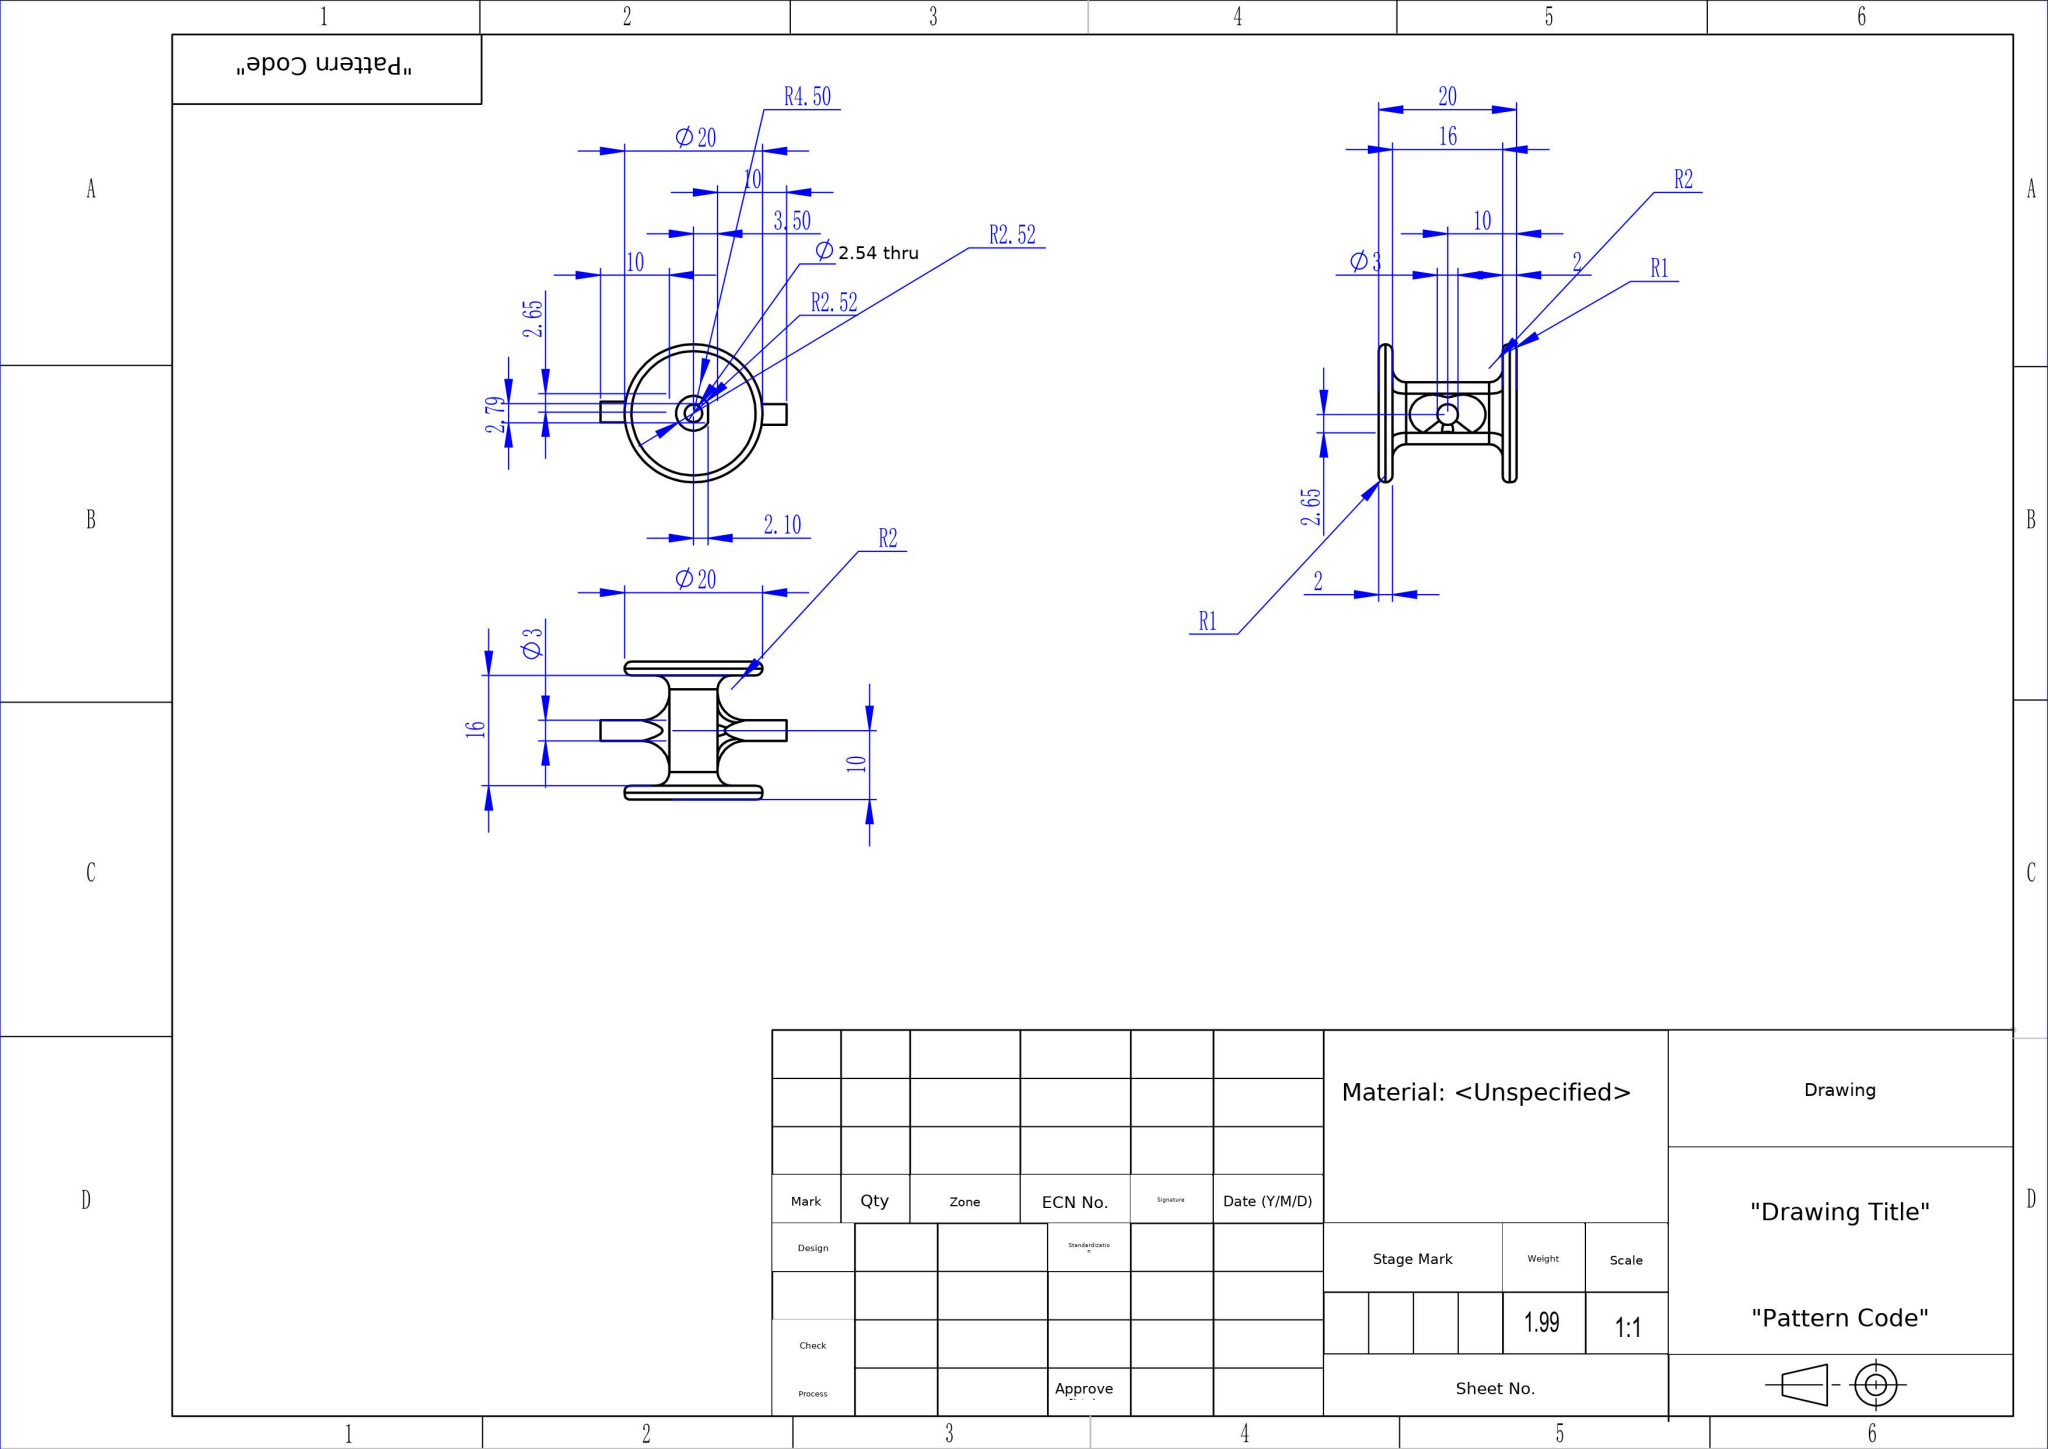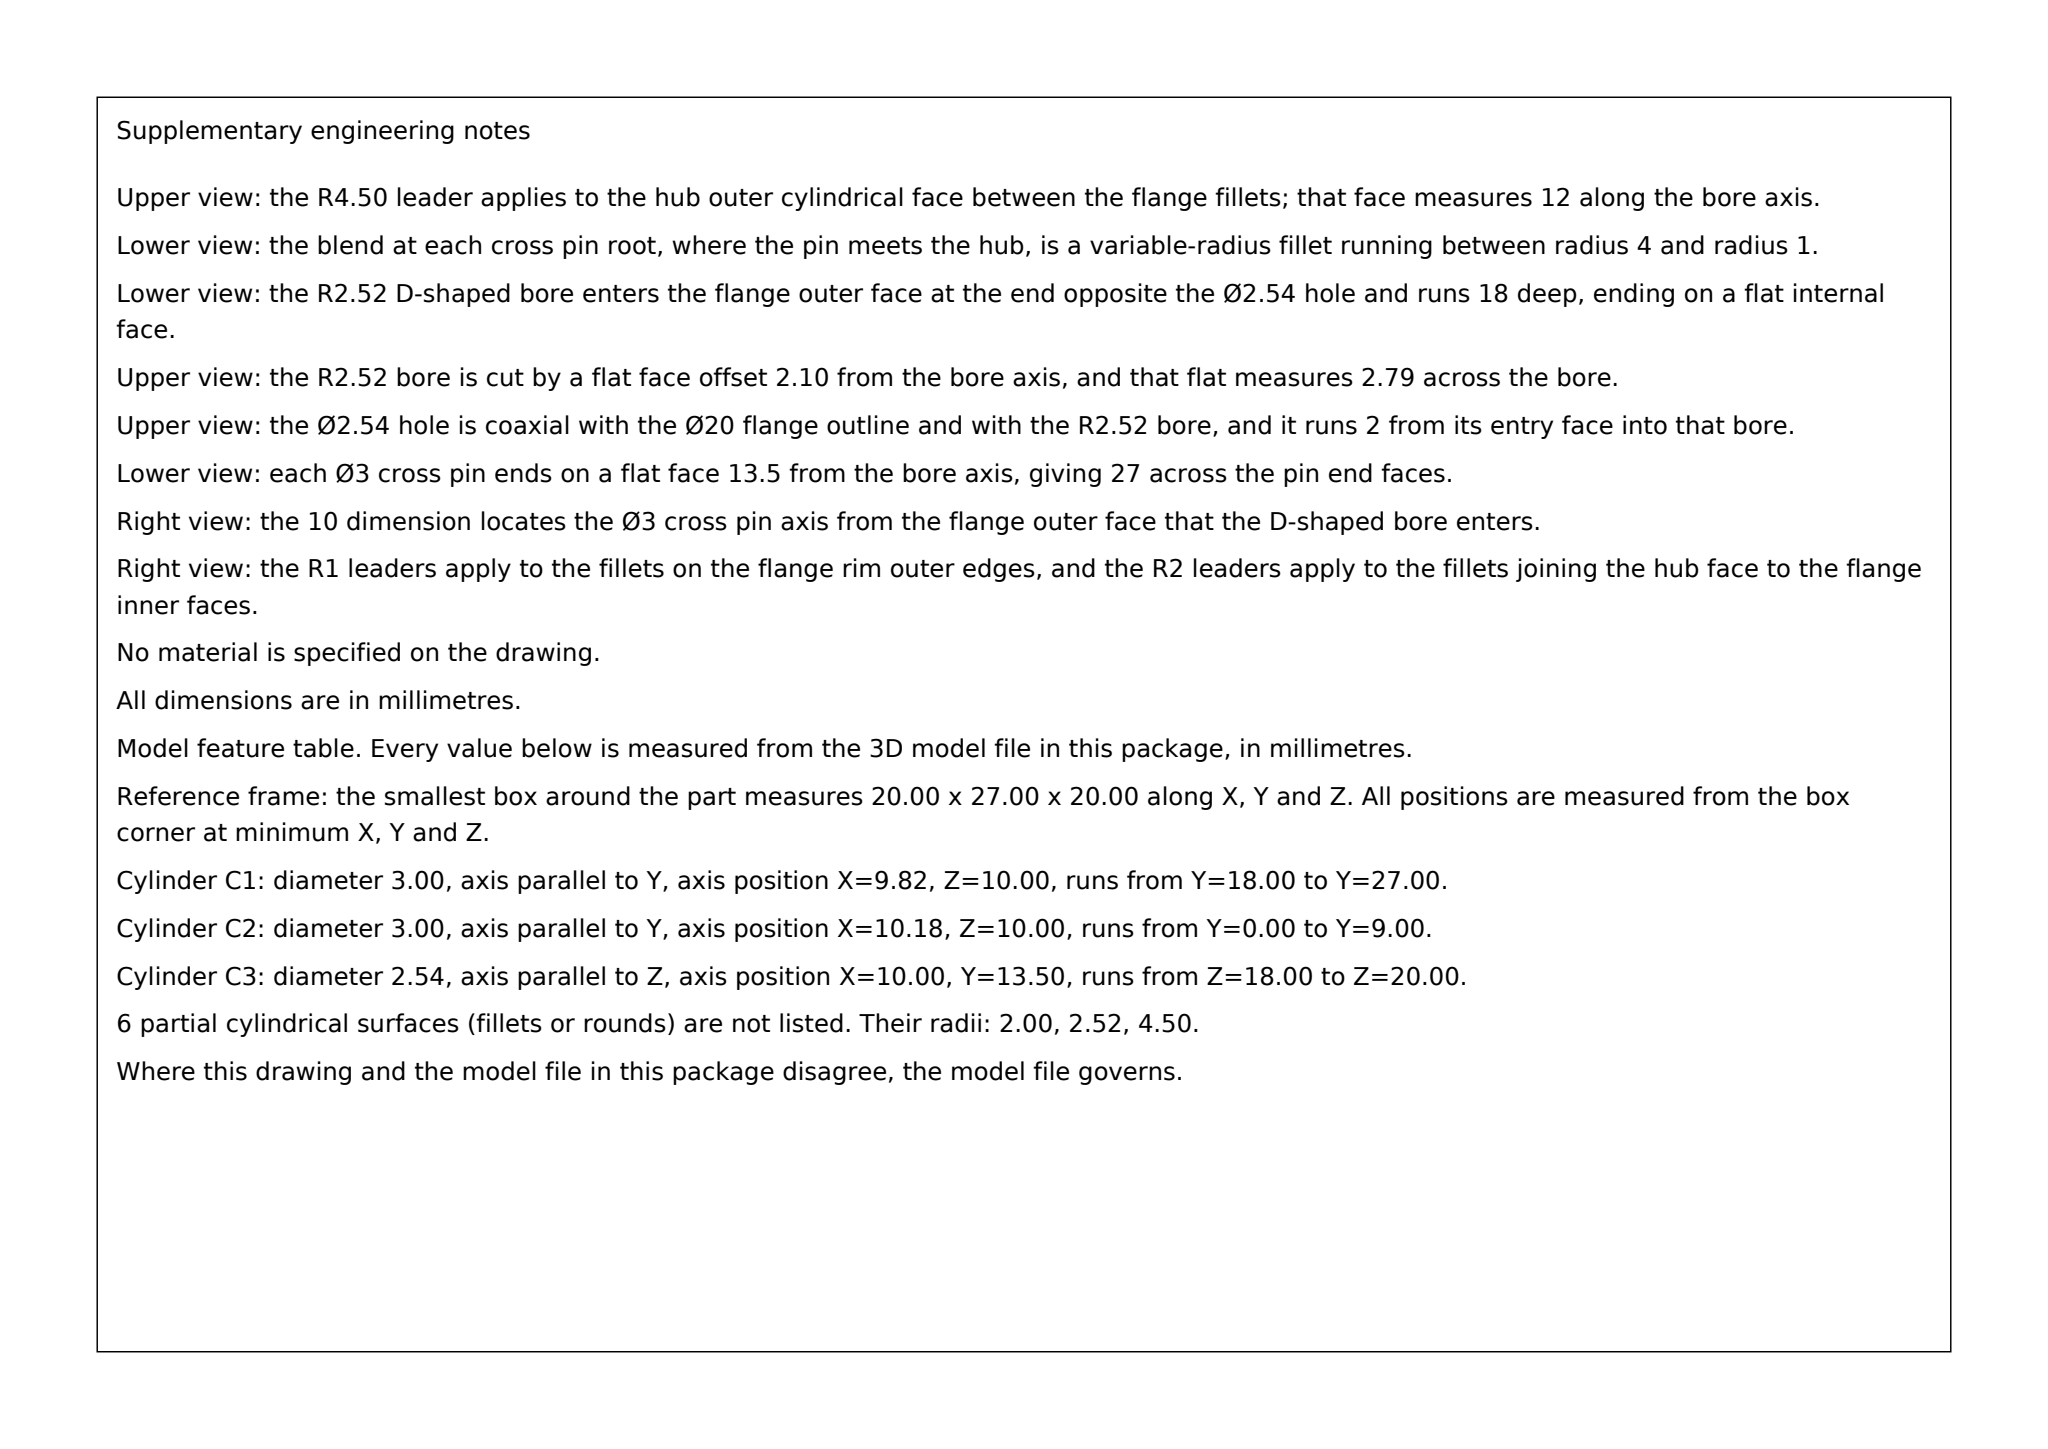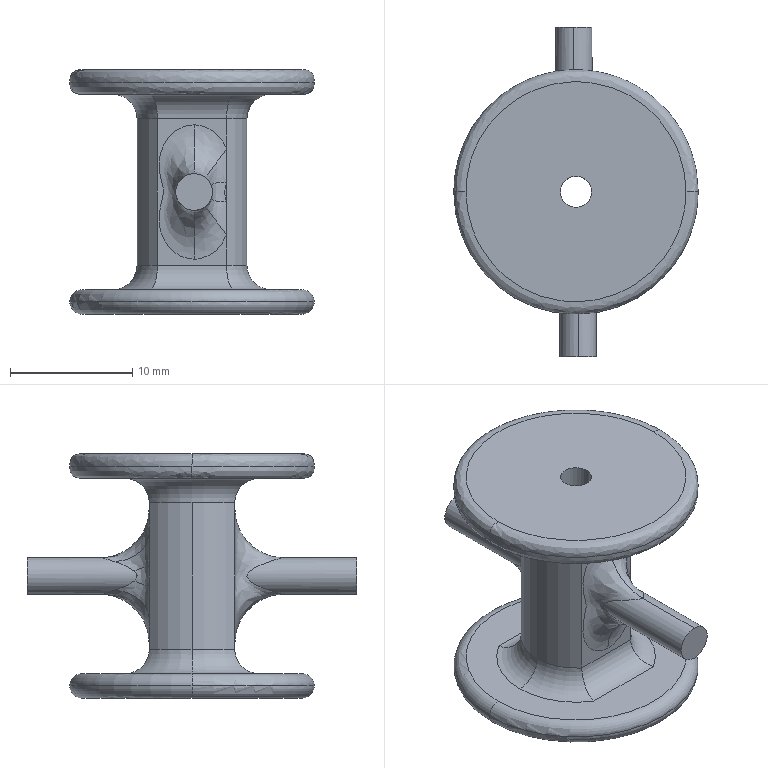Part | SolidWorks | mm | 1 solid | 54 faces | box 20 x 27 x 20 mm | volume 1989 mm3 | spline 16 | cylinder 16 | plane 12 | torus 10 | commonest cylinder face diameters 3 x4 4 x4 5.04 x3 9 x3 2.544 x2
Drawing notes:
CENTER HOLE Ø5.04 DEEP 18, AXIS AT X=10.82, Y=13.5 FROM BBOX MIN CORNER (replaces garbled '11 18 DEEP' callout) | from the solid: cylinders: [5.04,"z",[10.82,13.5,null],18.0]
COUNTERBORE / INTERNAL BORE Ø9 DEEP 12, COAXIAL WITH Ø5.04 HOLE AT X=10.82, Y=13.5 | from the solid: cylinders: [9.0,"z",[10.82,13.5,null],12.0]
2X Ø2.54 THRU 2 THK END LAND (Z=0 TO 2 AND Z=18 TO 20), COAXIAL WITH Ø9 BORE AT X=10.82, Y=13.5 | from the solid: cylinders: [2.544,"z",[10.82,13.5,null],2.0,count 2]; axis_planes z=0,2,18,20
4X Ø4 x 6.93 LG SIDE BOSSES, AXIS PARALLEL TO X, AT Y=8 AND Y=19, Z=4 AND Z=16 FROM BBOX MIN CORNER | from the solid: cylinders: [4.0,"x",[null,8.0,4.0],6.93], [4.0,"x",[null,8.0,16.0],6.93], [4.0,"x",[null,19.0,4.0],6.93], [4.0,"x",[null,19.0,16.0],6.93]
OVERALL WIDTH ACROSS SIDE BOSSES 21.65 (X DIRECTION) | from the solid: bbox_xyz X = 21.649
4X Ø3 CROSS HOLES, AXIS PARALLEL TO Y, LOCATED Z=10 FROM BOTTOM FACE (Z=0), X=10.64 AND X=11.00, 9 LG EACH | from the solid: cylinders: [3.0,"y",[10.64,null,10.0],9.0,2] and [3.0,"y",[11.0,null,10.0],9.0,2]
R4 FEATURE IS GROOVE FILLET R2 (6 PLACES) AND R1 (4 PLACES) - replaces garbled '22 R4' callout | from the solid: fillet_radii: [[1.0,4],[2.0,6]]
ALL DIMENSIONS IN MILLIMETERS | from the solid: STEP model facts stated in mm
CENTRAL BORE: Ø5.04, 18 DEEP, ON SPOOL AXIS AT X=10.82 / Y=13.50 FROM BBOX MIN CORNER (replaces garbled '11 18 DEEP' callout) | from the solid: cylinders: [5.04,"z",[10.82,13.5],18.0]
COUNTERBORE Ø9 x 12 DEEP, COAXIAL WITH Ø5.04 BORE, AXIS AT X=10.82 / Y=13.50 | from the solid: cylinders: [9.0,"z",[10.82,13.5],12.0]
4X Ø4 CROSS HOLES, AXIS PARALLEL TO X, LENGTH 6.93 EACH, AT Y=8 AND Y=19, Z=4 AND Z=16 FROM BBOX MIN CORNER | from the solid: cylinders: [4.0,"x",[null,8,4],6.93], [4.0,"x",[null,8,16],6.93], [4.0,"x",[null,19,4],6.93], [4.0,"x",[null,19,16],6.93]
OVERALL WIDTH ACROSS SIDE LUGS = 21.65 (X DIRECTION) | from the solid: bbox_xyz X = 21.649
OVERALL HEIGHT 27.00 (Y) x 20.00 (Z) ENVELOPE | from the solid: bbox_xyz = [21.649, 27.001, 20.001]
2X Ø2.54 THRU FEATURE, 2 DEEP LAND EACH END, AXIS AT X=10.82 / Y=13.50; LAND FACES AT Z=0 TO Z=2 AND Z=18 TO Z=20 | from the solid: cylinders: [2.544,"z",[10.82,13.5],2.0,2]; axis_planes z=0, z=2, z=18, z=20
Ø3 CROSS HOLES, AXIS PARALLEL TO Y, LOCATED AT Z=10.00 FROM BBOX MIN CORNER, LENGTH 9 EACH, AT X=10.64 AND X=11.00 | from the solid: cylinders: [3.0,"y",[10.64,null,10.0],9.0,2] and [3.0,"y",[11.0,null,10.0],9.0,2]
FILLETS: R2 (6 PLACES) AND R1 (4 PLACES) UNLESS OTHERWISE NOTED (replaces garbled 'R4' callout) | from the solid: fillet_radii: [[1.0,4],[2.0,6]]
CENTER HOLE Ø5.04 DEEP 18, AXIS AT X=10.82, Y=13.50 FROM BBOX MIN CORNER (replaces garbled '11 18 DEEP') | from the solid: cylinders: [5.04,'z',[10.82,13.5],18.0]
COUNTERBORE Ø9 DEEP 12, COAXIAL WITH Ø5.04 HOLE AT X=10.82, Y=13.50 | from the solid: cylinders: [9.0,'z',[10.82,13.5],12.0]
4X Ø4 CROSS BOSS/HOLE, LENGTH 6.93 ALONG X, AXES AT (Y=8, Z=4), (Y=8, Z=16), (Y=19, Z=4), (Y=19, Z=16) FROM BBOX MIN CORNER | from the solid: cylinders: [4.0,'x',[null,8.0,4.0],6.93] / [4.0,'x',[null,8.0,16.0],6.93] / [4.0,'x',[null,19.0,4.0],6.93] / [4.0,'x',[null,19.0,16.0],6.93]
OVERALL WIDTH ACROSS SIDE LUGS = 21.65 (X EXTENT) | from the solid: bbox_xyz X = 21.649
Ø2.54 THRU FEATURE: 2 LAND AT EACH END FACE (Z=0 TO 2 AND Z=18 TO 20), AXIS AT X=10.82, Y=13.50 FROM BBOX MIN CORNER | from the solid: cylinders: [2.544,'z',[10.82,13.5],2.0,count 2]; axis_planes z=0,2,18,20
Ø3 CROSS HOLES, AXES ALONG Y, LENGTH 9, LOCATED AT Z=10 FROM BBOX MIN CORNER (X=10.64 AND X=11.00) | from the solid: cylinders: [3.0,'y',[10.64,null,10.0],9.0] and [3.0,'y',[11.0,null,10.0],9.0]
FLATS: PLANAR FACES NORMAL TO Y AT Y=10.00 (2 PLACES), Y=15.60 (1 PLACE) AND Y=17.00 (2 PLACES) FROM BBOX MIN CORNER; BOUNDING FACES AT Y=0 AND Y=27.00 (27.00 OVERALL Y) | from the solid: axis_planes normal y at 0.0, 10.0 (x2), 15.6, 17.0 (x2), 27.0; bbox_xyz Y=27.001
END LAND FACES NORMAL TO Z AT Z=0, Z=2.00, Z=18.00 AND Z=20.00 FROM BBOX MIN CORNER (2 THK LAND EACH END) | from the solid: axis_planes normal z at 0.0, 2.0, 18.0, 20.0; cylinder dia 2.544 axis z length 2.0
CENTER BORE Ø5.04 DEEP 18 WITH Ø9 COUNTERBORE DEEP 12, AXIS AT X=10.82 / Y=13.50 FROM BBOX MIN CORNER (replaces redacted garbled callout) | from the solid: cylinders dia 5.04 axis z at (10.82,13.5) length 18; dia 9.0 axis z at (10.82,13.5) length 12
ALL FILLETS R2 (6 PLACES) AND R1 (4 PLACES) UNLESS OTHERWISE NOTED (replaces redacted garbled callout) | from the solid: fillet_radii [[1.0,4],[2.0,6]]
SPOOL GROOVE ROOT (CORE) Ø9 CYLINDRICAL, FROM Z=4.00 TO Z=16.00 (12 WIDE) BETWEEN FLANGE INNER FACES, AXIS AT X=10.82 / Y=13.50 FROM BBOX MIN CORNER | from the solid: cylinders: convex arc (round/outer radius) dia 9.0, axis z at [10.8,13.5], from 4.0 to 16.0
GROOVE PROFILE: Ø9 ROOT BLENDED TO Ø20 FLANGES BY R2 FILLETS (TORUS MAJOR R6.5); FLANGE OUTER EDGES R1 (TORUS MAJOR R9) | from the solid: tori: [minor_r 2.0, major 6.5, 6 places] and [minor_r 1.0, major 9.0, 4 places]
CENTER HOLE Ø5.04 DEEP 18 FROM Z=0, AXIS AT X=10.82 / Y=13.50 FROM BBOX MIN CORNER (replaces redacted garbled callout) | from the solid: cylinders: concave arc dia 5.04, axis z at [10.8,13.5], from 0.0 to 18.0